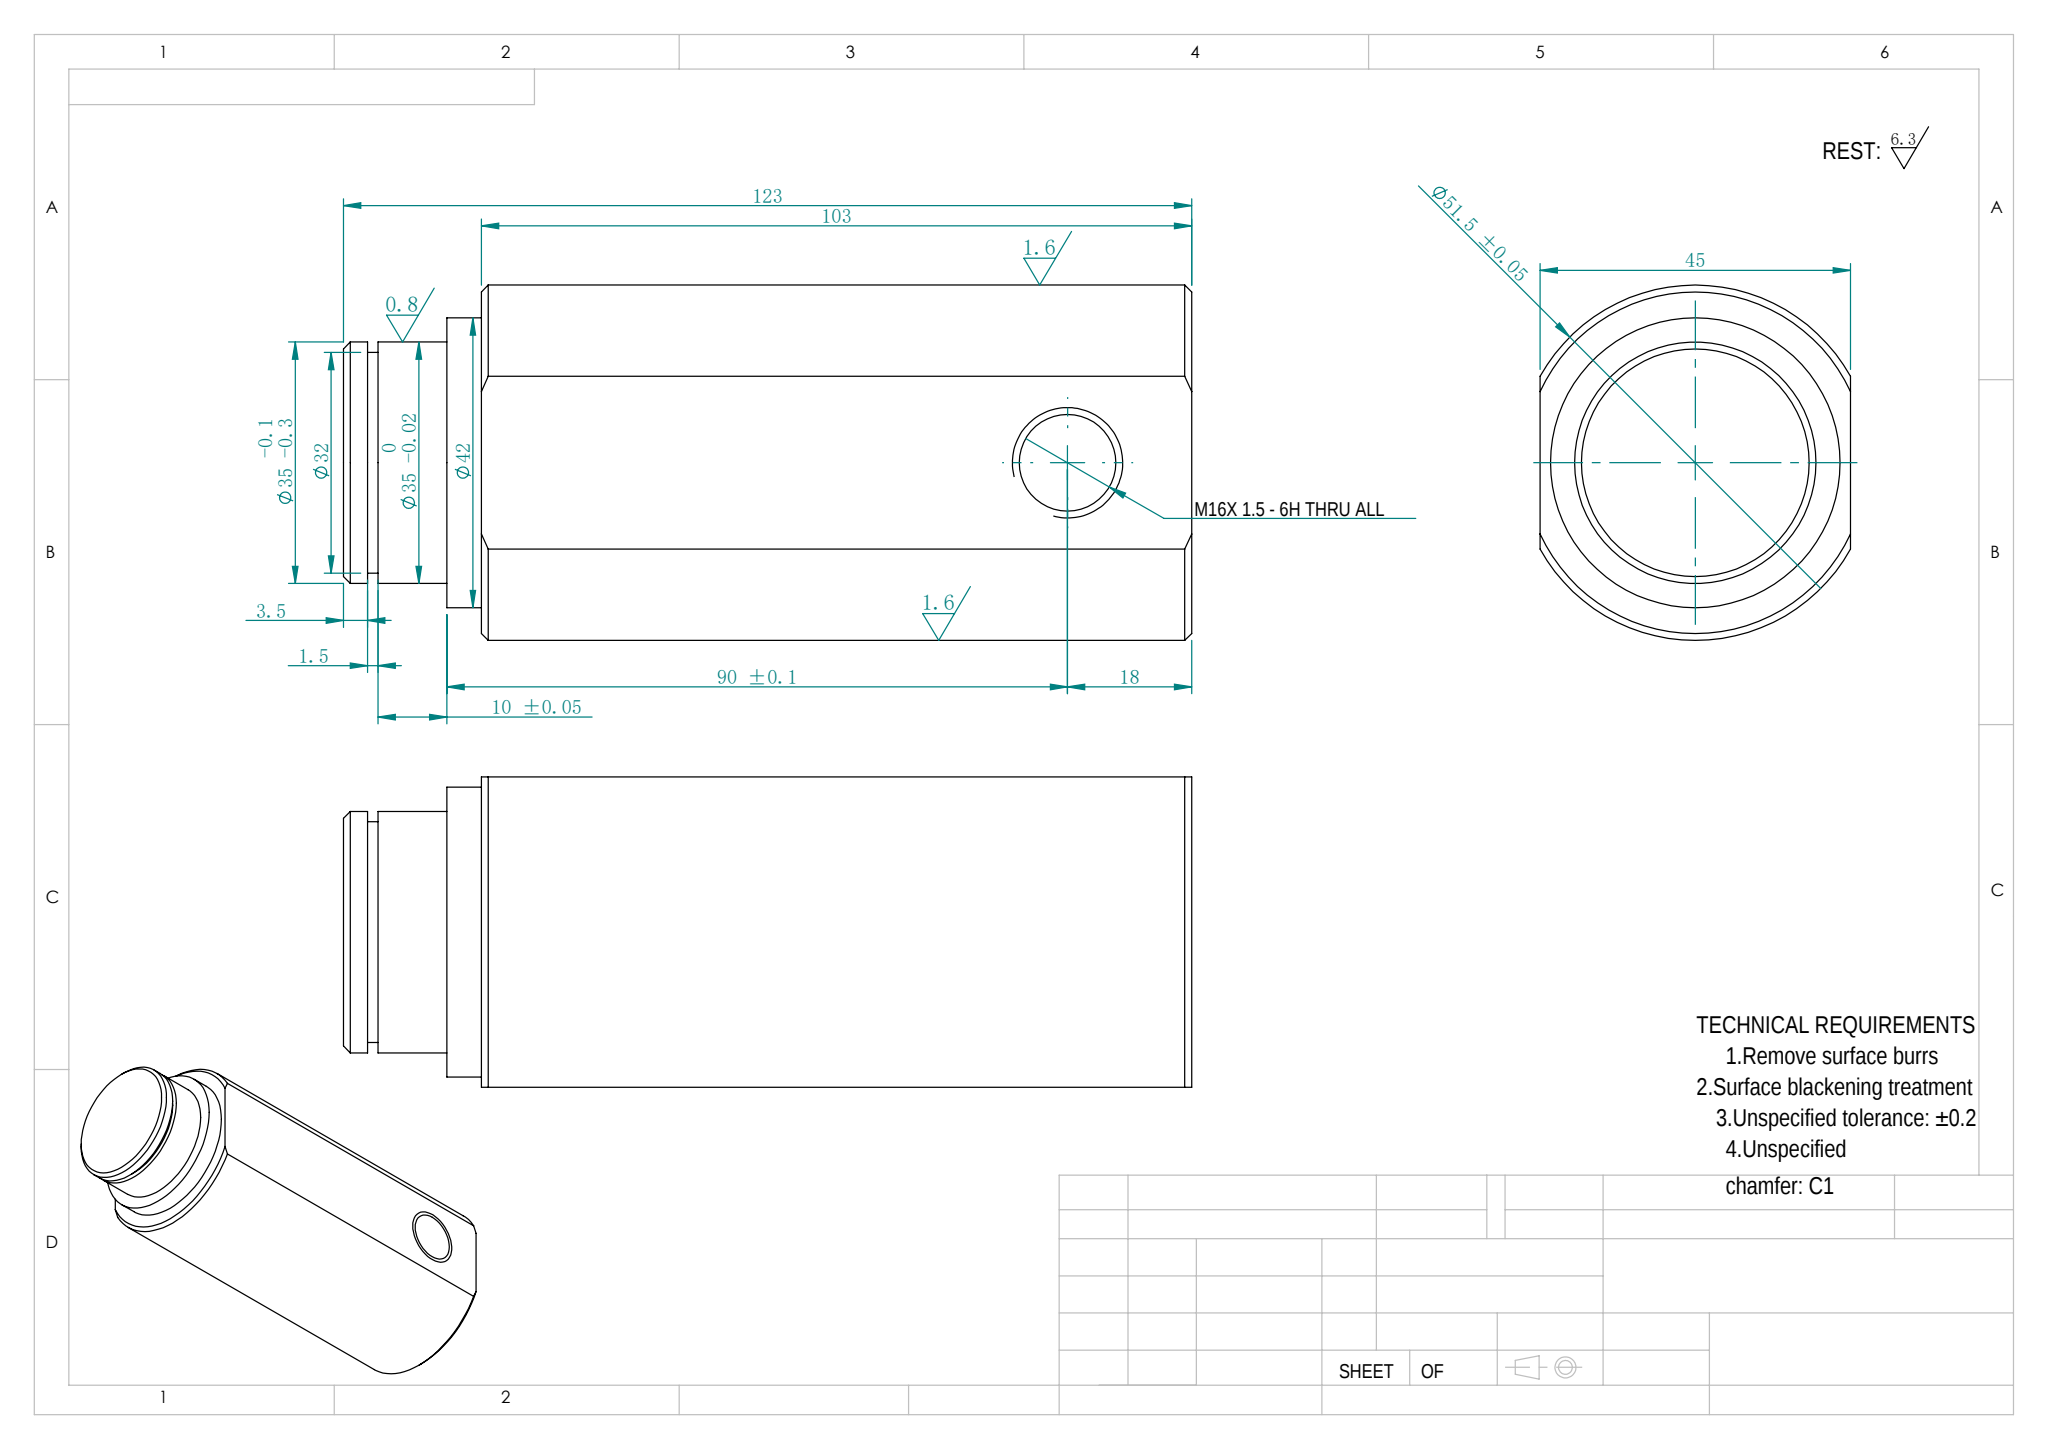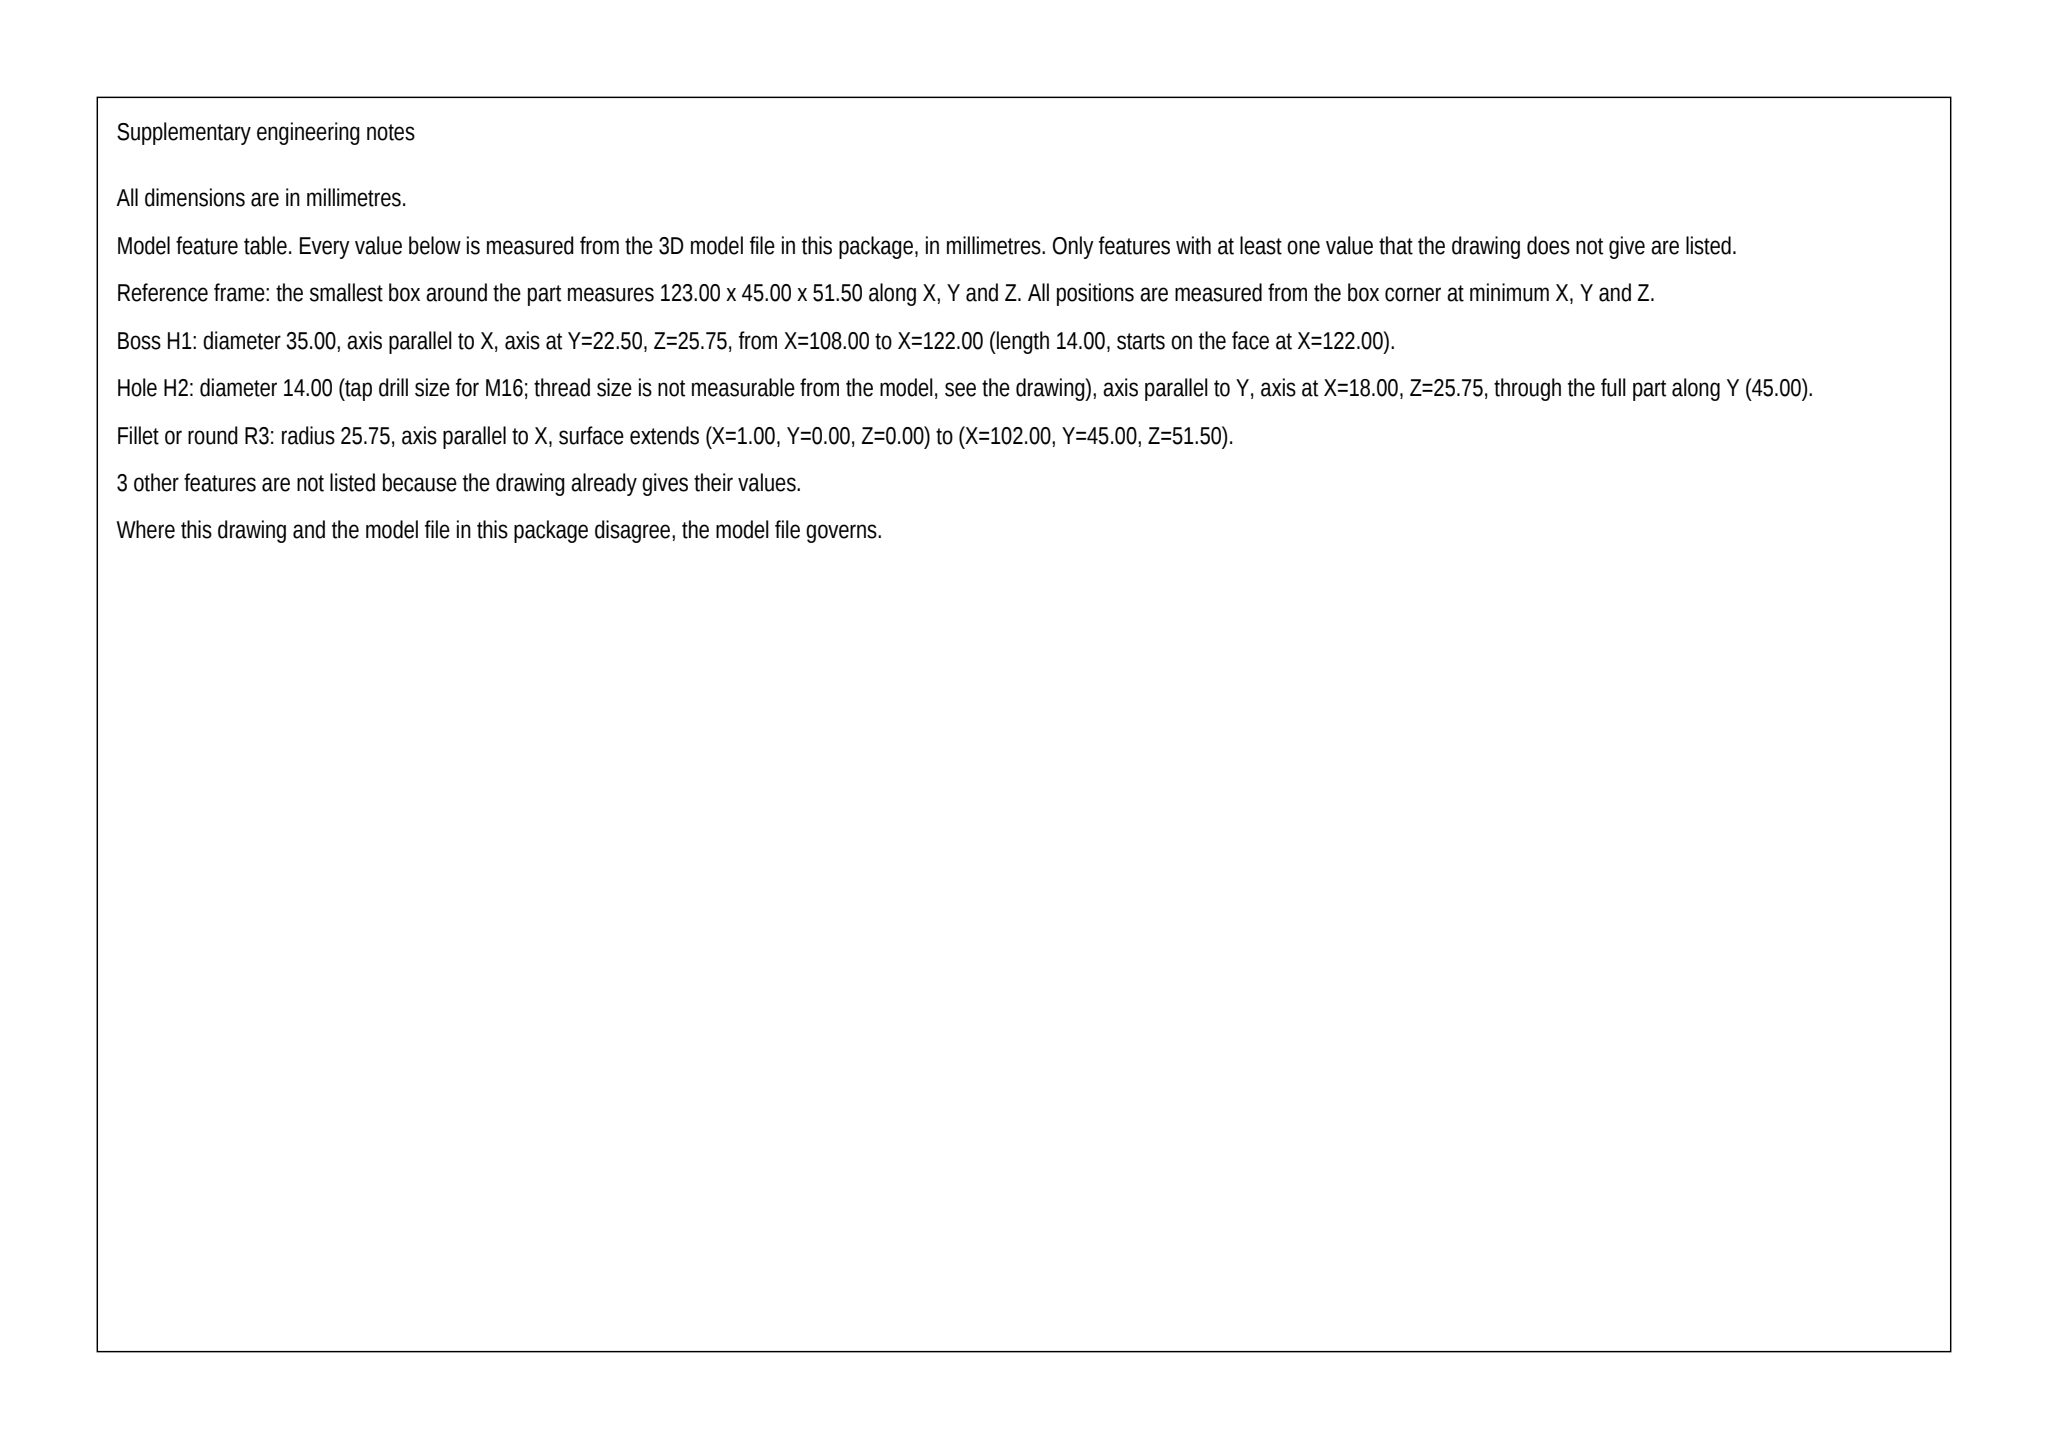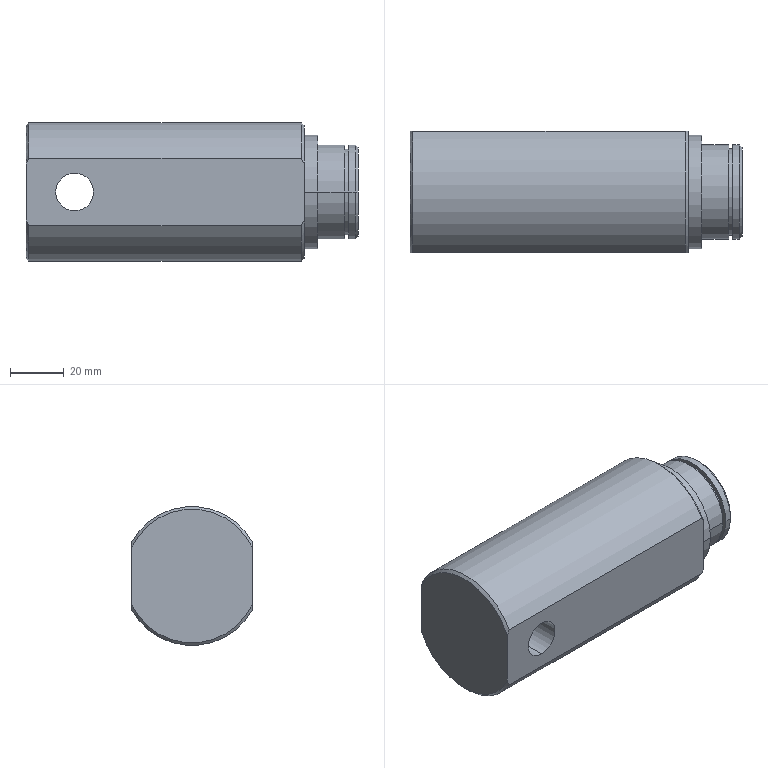Part | SolidWorks | mm | 1 solid | 26 faces | box 123 x 45 x 51.5 mm | volume 217259 mm3 | cylinder 12 | plane 8 | cone 6 | commonest cylinder face diameters 35 x4 14 x2 32 x2 42 x2 51.5 x2
build123d program:
from build123d import *

# Parameters (mm, degrees)
SKETCH2_OUTSIDE_W   = 82.09
SKETCH2_OUTSIDE_H   = 82.09
SKETCH2_OUTSIDE_W_2 = 65
SKETCH2_OUTSIDE_H_2 = 45
CUT_EXTRUDE1_DEPTH  = 129.278
M16_TAPPED_HOLE1_D  = 14
CHAMFER1_SIZE       = 1


with BuildPart() as part:
    # Sketch1 → Revolve1 (revolve)
    with BuildSketch(Plane.XY):
        Polygon((0, 0), (0, 25.75), (103, 25.75), (103, 21), (108, 21), (108, 17.5), (118, 17.5), (118, 16), (119.5, 16), (119.5, 17.5), (123, 17.5), (123, 0), align=None)
    revolve(axis=Axis((123, 0, 0), (-1, 0, 0)))

    # Sketch2 outside → Cut-Extrude1 (cut, through all)
    with BuildSketch(Plane.ZY):
        Rectangle(SKETCH2_OUTSIDE_W, SKETCH2_OUTSIDE_H)
        Rectangle(SKETCH2_OUTSIDE_W_2, SKETCH2_OUTSIDE_H_2, mode=Mode.SUBTRACT)
    extrude(amount=-CUT_EXTRUDE1_DEPTH, mode=Mode.SUBTRACT)

    # M16 Tapped Hole1 (through all)
    with Locations(Plane(origin=(0, 22.5, 0), x_dir=(1, 0, 0), z_dir=(0, 1, 0))):
        with Locations((18, 0)):
            Hole(M16_TAPPED_HOLE1_D / 2)

    # Chamfer1
    chamfer1_edges = [part.edges().sort_by_distance(p)[0] for p in [
        (103, 0, 25.75),
        (0, 0, 25.75),
        (103, 0, -25.75),
        (0, 0, -25.75),
        (123, -17.5, 0),
    ]]
    chamfer(chamfer1_edges, length=CHAMFER1_SIZE)


solid = part.part
STEP:
#1=CARTESIAN_POINT('',(123.,16.5,0.));
#2=VERTEX_POINT('',#1);
#3=CARTESIAN_POINT('',(123.,-16.5,0.));
#4=VERTEX_POINT('',#3);
#5=CARTESIAN_POINT('',(123.,0.,0.));
#6=DIRECTION('',(1.,0.,0.));
#7=DIRECTION('',(0.,1.,0.));
#8=AXIS2_PLACEMENT_3D('',#5,#6,#7);
#9=CIRCLE('',#8,16.5);
#10=EDGE_CURVE('',#2,#4,#9,.T.);
#11=ORIENTED_EDGE('',*,*,#10,.F.);
#12=CARTESIAN_POINT('',(122.,17.5,0.));
#13=VERTEX_POINT('',#12);
#14=CARTESIAN_POINT('',(123.,16.5,0.));
#15=DIRECTION('',(-0.7071,0.7071,0.));
#16=VECTOR('',#15,1000.);
#17=LINE('',#14,#16);
#18=EDGE_CURVE('',#2,#13,#17,.T.);
#19=ORIENTED_EDGE('',*,*,#18,.T.);
#20=CARTESIAN_POINT('',(122.,-17.5,0.));
#21=VERTEX_POINT('',#20);
#22=CARTESIAN_POINT('',(122.,0.,0.));
#23=DIRECTION('',(-1.,-0.,0.));
#24=DIRECTION('',(0.,1.,0.));
#25=AXIS2_PLACEMENT_3D('',#22,#23,#24);
#26=CIRCLE('',#25,17.5);
#27=EDGE_CURVE('',#21,#13,#26,.T.);
#28=ORIENTED_EDGE('',*,*,#27,.F.);
#29=CARTESIAN_POINT('',(123.,-16.5,0.));
#30=DIRECTION('',(-0.7071,-0.7071,0.));
#31=VECTOR('',#30,1000.);
#32=LINE('',#29,#31);
#33=EDGE_CURVE('',#4,#21,#32,.T.);
#34=ORIENTED_EDGE('',*,*,#33,.F.);
#35=EDGE_LOOP('',(#11,#19,#28,#34));
#36=FACE_OUTER_BOUND('',#35,.T.);
#37=CARTESIAN_POINT('',(123.,0.,0.));
#38=DIRECTION('',(-1.,-0.,0.));
#39=DIRECTION('',(0.,-1.,0.));
#40=AXIS2_PLACEMENT_3D('',#37,#38,#39);
#41=CONICAL_SURFACE('',#40,16.5,0.7854);
#42=ADVANCED_FACE('',(#36),#41,.T.);
#43=CARTESIAN_POINT('',(18.,-22.5,-7.));
#44=VERTEX_POINT('',#43);
#45=CARTESIAN_POINT('',(18.,-22.5,7.));
#46=VERTEX_POINT('',#45);
#47=CARTESIAN_POINT('',(18.,-22.5,0.));
#48=DIRECTION('',(0.,1.,0.));
#49=DIRECTION('',(0.,0.,1.));
#50=AXIS2_PLACEMENT_3D('',#47,#48,#49);
#51=CIRCLE('',#50,7.);
#52=EDGE_CURVE('',#44,#46,#51,.T.);
#53=ORIENTED_EDGE('',*,*,#52,.F.);
#54=CARTESIAN_POINT('',(18.,22.5,-7.));
#55=VERTEX_POINT('',#54);
#56=CARTESIAN_POINT('',(18.,22.5,-7.));
#57=DIRECTION('',(0.,1.,0.));
#58=VECTOR('',#57,1000.);
#59=LINE('',#56,#58);
#60=EDGE_CURVE('',#44,#55,#59,.T.);
#61=ORIENTED_EDGE('',*,*,#60,.T.);
#62=CARTESIAN_POINT('',(18.,22.5,7.));
#63=VERTEX_POINT('',#62);
#64=CARTESIAN_POINT('',(18.,22.5,0.));
#65=DIRECTION('',(0.,1.,0.));
#66=DIRECTION('',(0.,0.,1.));
#67=AXIS2_PLACEMENT_3D('',#64,#65,#66);
#68=CIRCLE('',#67,7.);
#69=EDGE_CURVE('',#55,#63,#68,.T.);
#70=ORIENTED_EDGE('',*,*,#69,.T.);
#71=CARTESIAN_POINT('',(18.,22.5,7.));
#72=DIRECTION('',(0.,1.,0.));
#73=VECTOR('',#72,1000.);
#74=LINE('',#71,#73);
#75=EDGE_CURVE('',#46,#63,#74,.T.);
#76=ORIENTED_EDGE('',*,*,#75,.F.);
#77=EDGE_LOOP('',(#53,#61,#70,#76));
#78=FACE_OUTER_BOUND('',#77,.T.);
#79=CARTESIAN_POINT('',(18.,22.5,0.));
#80=DIRECTION('',(0.,1.,0.));
#81=DIRECTION('',(0.,0.,1.));
#82=AXIS2_PLACEMENT_3D('',#79,#80,#81);
#83=CYLINDRICAL_SURFACE('',#82,7.);
#84=ADVANCED_FACE('',(#78),#83,.F.);
#85=CARTESIAN_POINT('',(119.5,17.5,0.));
#86=VERTEX_POINT('',#85);
#87=CARTESIAN_POINT('',(119.5,-17.5,0.));
#88=VERTEX_POINT('',#87);
#89=CARTESIAN_POINT('',(119.5,0.,0.));
#90=DIRECTION('',(1.,0.,0.));
#91=DIRECTION('',(0.,1.,0.));
#92=AXIS2_PLACEMENT_3D('',#89,#90,#91);
#93=CIRCLE('',#92,17.5);
#94=EDGE_CURVE('',#86,#88,#93,.T.);
#95=ORIENTED_EDGE('',*,*,#94,.T.);
#96=CARTESIAN_POINT('',(123.,-17.5,0.));
#97=DIRECTION('',(1.,0.,0.));
#98=VECTOR('',#97,1000.);
#99=LINE('',#96,#98);
#100=EDGE_CURVE('',#88,#21,#99,.T.);
#101=ORIENTED_EDGE('',*,*,#100,.T.);
#102=ORIENTED_EDGE('',*,*,#27,.T.);
#103=CARTESIAN_POINT('',(123.,17.5,0.));
#104=DIRECTION('',(1.,0.,0.));
#105=VECTOR('',#104,1000.);
#106=LINE('',#103,#105);
#107=EDGE_CURVE('',#86,#13,#106,.T.);
#108=ORIENTED_EDGE('',*,*,#107,.F.);
#109=EDGE_LOOP('',(#95,#101,#102,#108));
#110=FACE_OUTER_BOUND('',#109,.T.);
#111=CARTESIAN_POINT('',(123.,0.,0.));
#112=DIRECTION('',(1.,0.,0.));
#113=DIRECTION('',(0.,1.,0.));
#114=AXIS2_PLACEMENT_3D('',#111,#112,#113);
#115=CYLINDRICAL_SURFACE('',#114,17.5);
#116=ADVANCED_FACE('',(#110),#115,.T.);
#117=CARTESIAN_POINT('',(118.,16.,0.));
#118=VERTEX_POINT('',#117);
#119=CARTESIAN_POINT('',(118.,-16.,0.));
#120=VERTEX_POINT('',#119);
#121=CARTESIAN_POINT('',(118.,0.,0.));
#122=DIRECTION('',(1.,0.,0.));
#123=DIRECTION('',(0.,1.,0.));
#124=AXIS2_PLACEMENT_3D('',#121,#122,#123);
#125=CIRCLE('',#124,16.);
#126=EDGE_CURVE('',#118,#120,#125,.T.);
#127=ORIENTED_EDGE('',*,*,#126,.T.);
#128=CARTESIAN_POINT('',(119.5,-16.,0.));
#129=VERTEX_POINT('',#128);
#130=CARTESIAN_POINT('',(123.,-16.,0.));
#131=DIRECTION('',(1.,0.,0.));
#132=VECTOR('',#131,1000.);
#133=LINE('',#130,#132);
#134=EDGE_CURVE('',#120,#129,#133,.T.);
#135=ORIENTED_EDGE('',*,*,#134,.T.);
#136=CARTESIAN_POINT('',(119.5,16.,0.));
#137=VERTEX_POINT('',#136);
#138=CARTESIAN_POINT('',(119.5,0.,0.));
#139=DIRECTION('',(1.,0.,0.));
#140=DIRECTION('',(0.,1.,0.));
#141=AXIS2_PLACEMENT_3D('',#138,#139,#140);
#142=CIRCLE('',#141,16.);
#143=EDGE_CURVE('',#137,#129,#142,.T.);
#144=ORIENTED_EDGE('',*,*,#143,.F.);
#145=CARTESIAN_POINT('',(123.,16.,0.));
#146=DIRECTION('',(1.,0.,0.));
#147=VECTOR('',#146,1000.);
#148=LINE('',#145,#147);
#149=EDGE_CURVE('',#118,#137,#148,.T.);
#150=ORIENTED_EDGE('',*,*,#149,.F.);
#151=EDGE_LOOP('',(#127,#135,#144,#150));
#152=FACE_OUTER_BOUND('',#151,.T.);
#153=CARTESIAN_POINT('',(123.,0.,0.));
#154=DIRECTION('',(1.,0.,0.));
#155=DIRECTION('',(0.,1.,0.));
#156=AXIS2_PLACEMENT_3D('',#153,#154,#155);
#157=CYLINDRICAL_SURFACE('',#156,16.);
#158=ADVANCED_FACE('',(#152),#157,.T.);
#159=CARTESIAN_POINT('',(108.,17.5,0.));
#160=VERTEX_POINT('',#159);
#161=CARTESIAN_POINT('',(108.,-17.5,0.));
#162=VERTEX_POINT('',#161);
#163=CARTESIAN_POINT('',(108.,0.,0.));
#164=DIRECTION('',(1.,0.,0.));
#165=DIRECTION('',(0.,1.,0.));
#166=AXIS2_PLACEMENT_3D('',#163,#164,#165);
#167=CIRCLE('',#166,17.5);
#168=EDGE_CURVE('',#160,#162,#167,.T.);
#169=ORIENTED_EDGE('',*,*,#168,.T.);
#170=CARTESIAN_POINT('',(118.,-17.5,0.));
#171=VERTEX_POINT('',#170);
#172=CARTESIAN_POINT('',(123.,-17.5,0.));
#173=DIRECTION('',(1.,0.,0.));
#174=VECTOR('',#173,1000.);
#175=LINE('',#172,#174);
#176=EDGE_CURVE('',#162,#171,#175,.T.);
#177=ORIENTED_EDGE('',*,*,#176,.T.);
#178=CARTESIAN_POINT('',(118.,17.5,0.));
#179=VERTEX_POINT('',#178);
#180=CARTESIAN_POINT('',(118.,0.,0.));
#181=DIRECTION('',(1.,0.,0.));
#182=DIRECTION('',(0.,1.,0.));
#183=AXIS2_PLACEMENT_3D('',#180,#181,#182);
#184=CIRCLE('',#183,17.5);
#185=EDGE_CURVE('',#179,#171,#184,.T.);
#186=ORIENTED_EDGE('',*,*,#185,.F.);
#187=CARTESIAN_POINT('',(123.,17.5,0.));
#188=DIRECTION('',(1.,0.,0.));
#189=VECTOR('',#188,1000.);
#190=LINE('',#187,#189);
#191=EDGE_CURVE('',#160,#179,#190,.T.);
#192=ORIENTED_EDGE('',*,*,#191,.F.);
#193=EDGE_LOOP('',(#169,#177,#186,#192));
#194=FACE_OUTER_BOUND('',#193,.T.);
#195=CARTESIAN_POINT('',(123.,0.,0.));
#196=DIRECTION('',(1.,0.,0.));
#197=DIRECTION('',(0.,1.,0.));
#198=AXIS2_PLACEMENT_3D('',#195,#196,#197);
#199=CYLINDRICAL_SURFACE('',#198,17.5);
#200=ADVANCED_FACE('',(#194),#199,.T.);
#201=CARTESIAN_POINT('',(103.,21.,0.));
#202=VERTEX_POINT('',#201);
#203=CARTESIAN_POINT('',(103.,-21.,0.));
#204=VERTEX_POINT('',#203);
#205=CARTESIAN_POINT('',(103.,0.,0.));
#206=DIRECTION('',(1.,0.,0.));
#207=DIRECTION('',(0.,1.,0.));
#208=AXIS2_PLACEMENT_3D('',#205,#206,#207);
#209=CIRCLE('',#208,21.);
#210=EDGE_CURVE('',#202,#204,#209,.T.);
#211=ORIENTED_EDGE('',*,*,#210,.T.);
#212=CARTESIAN_POINT('',(108.,-21.,0.));
#213=VERTEX_POINT('',#212);
#214=CARTESIAN_POINT('',(123.,-21.,0.));
#215=DIRECTION('',(1.,0.,0.));
#216=VECTOR('',#215,1000.);
#217=LINE('',#214,#216);
#218=EDGE_CURVE('',#204,#213,#217,.T.);
#219=ORIENTED_EDGE('',*,*,#218,.T.);
#220=CARTESIAN_POINT('',(108.,21.,0.));
#221=VERTEX_POINT('',#220);
#222=CARTESIAN_POINT('',(108.,0.,0.));
#223=DIRECTION('',(1.,0.,0.));
#224=DIRECTION('',(0.,1.,0.));
#225=AXIS2_PLACEMENT_3D('',#222,#223,#224);
#226=CIRCLE('',#225,21.);
#227=EDGE_CURVE('',#221,#213,#226,.T.);
#228=ORIENTED_EDGE('',*,*,#227,.F.);
#229=CARTESIAN_POINT('',(123.,21.,0.));
#230=DIRECTION('',(1.,0.,0.));
#231=VECTOR('',#230,1000.);
#232=LINE('',#229,#231);
#233=EDGE_CURVE('',#202,#221,#232,.T.);
#234=ORIENTED_EDGE('',*,*,#233,.F.);
#235=EDGE_LOOP('',(#211,#219,#228,#234));
#236=FACE_OUTER_BOUND('',#235,.T.);
#237=CARTESIAN_POINT('',(123.,0.,0.));
#238=DIRECTION('',(1.,0.,0.));
#239=DIRECTION('',(0.,1.,0.));
#240=AXIS2_PLACEMENT_3D('',#237,#238,#239);
#241=CYLINDRICAL_SURFACE('',#240,21.);
#242=ADVANCED_FACE('',(#236),#241,.T.);
#243=CARTESIAN_POINT('',(0.,-22.5,-10.311));
#244=VERTEX_POINT('',#243);
#245=CARTESIAN_POINT('',(0.,-22.5,10.311));
#246=VERTEX_POINT('',#245);
#247=CARTESIAN_POINT('',(0.,-22.5,-32.5));
#248=DIRECTION('',(0.,0.,1.));
#249=VECTOR('',#248,1000.);
#250=LINE('',#247,#249);
#251=EDGE_CURVE('',#244,#246,#250,.T.);
#252=ORIENTED_EDGE('',*,*,#251,.T.);
#253=CARTESIAN_POINT('',(-0.,22.5,10.311));
#254=VERTEX_POINT('',#253);
#255=CARTESIAN_POINT('',(0.,0.,0.));
#256=DIRECTION('',(-1.,-0.,0.));
#257=DIRECTION('',(0.,-1.,0.));
#258=AXIS2_PLACEMENT_3D('',#255,#256,#257);
#259=CIRCLE('',#258,24.75);
#260=EDGE_CURVE('',#246,#254,#259,.T.);
#261=ORIENTED_EDGE('',*,*,#260,.T.);
#262=CARTESIAN_POINT('',(-0.,22.5,-10.311));
#263=VERTEX_POINT('',#262);
#264=CARTESIAN_POINT('',(-0.,22.5,-32.5));
#265=DIRECTION('',(0.,0.,-1.));
#266=VECTOR('',#265,1000.);
#267=LINE('',#264,#266);
#268=EDGE_CURVE('',#254,#263,#267,.T.);
#269=ORIENTED_EDGE('',*,*,#268,.T.);
#270=CARTESIAN_POINT('',(0.,0.,0.));
#271=DIRECTION('',(-1.,-0.,0.));
#272=DIRECTION('',(0.,-1.,0.));
#273=AXIS2_PLACEMENT_3D('',#270,#271,#272);
#274=CIRCLE('',#273,24.75);
#275=EDGE_CURVE('',#263,#244,#274,.T.);
#276=ORIENTED_EDGE('',*,*,#275,.T.);
#277=EDGE_LOOP('',(#252,#261,#269,#276));
#278=FACE_OUTER_BOUND('',#277,.T.);
#279=CARTESIAN_POINT('',(0.,0.,0.));
#280=DIRECTION('',(-1.,-0.,0.));
#281=DIRECTION('',(0.,-1.,0.));
#282=AXIS2_PLACEMENT_3D('',#279,#280,#281);
#283=PLANE('',#282);
#284=ADVANCED_FACE('',(#278),#283,.T.);
#285=CARTESIAN_POINT('',(102.,-22.5,-12.522));
#286=VERTEX_POINT('',#285);
#287=CARTESIAN_POINT('',(1.,-22.5,-12.522));
#288=VERTEX_POINT('',#287);
#289=CARTESIAN_POINT('',(123.,-22.5,-12.522));
#290=DIRECTION('',(-1.,-0.,0.));
#291=VECTOR('',#290,1000.);
#292=LINE('',#289,#291);
#293=EDGE_CURVE('',#286,#288,#292,.T.);
#294=ORIENTED_EDGE('',*,*,#293,.T.);
#295=CARTESIAN_POINT('',(1.,22.5,-12.522));
#296=VERTEX_POINT('',#295);
#297=CARTESIAN_POINT('',(1.,0.,0.));
#298=DIRECTION('',(1.,0.,0.));
#299=DIRECTION('',(0.,-1.,0.));
#300=AXIS2_PLACEMENT_3D('',#297,#298,#299);
#301=CIRCLE('',#300,25.75);
#302=EDGE_CURVE('',#288,#296,#301,.T.);
#303=ORIENTED_EDGE('',*,*,#302,.T.);
#304=CARTESIAN_POINT('',(102.,22.5,-12.522));
#305=VERTEX_POINT('',#304);
#306=CARTESIAN_POINT('',(123.,22.5,-12.522));
#307=DIRECTION('',(1.,0.,0.));
#308=VECTOR('',#307,1000.);
#309=LINE('',#306,#308);
#310=EDGE_CURVE('',#296,#305,#309,.T.);
#311=ORIENTED_EDGE('',*,*,#310,.T.);
#312=CARTESIAN_POINT('',(102.,0.,0.));
#313=DIRECTION('',(-1.,-0.,0.));
#314=DIRECTION('',(0.,1.,0.));
#315=AXIS2_PLACEMENT_3D('',#312,#313,#314);
#316=CIRCLE('',#315,25.75);
#317=EDGE_CURVE('',#305,#286,#316,.T.);
#318=ORIENTED_EDGE('',*,*,#317,.T.);
#319=EDGE_LOOP('',(#294,#303,#311,#318));
#320=FACE_OUTER_BOUND('',#319,.T.);
#321=CARTESIAN_POINT('',(123.,0.,0.));
#322=DIRECTION('',(1.,0.,0.));
#323=DIRECTION('',(0.,1.,0.));
#324=AXIS2_PLACEMENT_3D('',#321,#322,#323);
#325=CYLINDRICAL_SURFACE('',#324,25.75);
#326=ADVANCED_FACE('',(#320),#325,.T.);
#327=CARTESIAN_POINT('',(102.,22.5,12.522));
#328=VERTEX_POINT('',#327);
#329=CARTESIAN_POINT('',(1.,22.5,12.522));
#330=VERTEX_POINT('',#329);
#331=CARTESIAN_POINT('',(123.,22.5,12.522));
#332=DIRECTION('',(-1.,-0.,0.));
#333=VECTOR('',#332,1000.);
#334=LINE('',#331,#333);
#335=EDGE_CURVE('',#328,#330,#334,.T.);
#336=ORIENTED_EDGE('',*,*,#335,.T.);
#337=CARTESIAN_POINT('',(1.,-22.5,12.522));
#338=VERTEX_POINT('',#337);
#339=CARTESIAN_POINT('',(1.,0.,0.));
#340=DIRECTION('',(1.,0.,0.));
#341=DIRECTION('',(0.,-1.,0.));
#342=AXIS2_PLACEMENT_3D('',#339,#340,#341);
#343=CIRCLE('',#342,25.75);
#344=EDGE_CURVE('',#330,#338,#343,.T.);
#345=ORIENTED_EDGE('',*,*,#344,.T.);
#346=CARTESIAN_POINT('',(102.,-22.5,12.522));
#347=VERTEX_POINT('',#346);
#348=CARTESIAN_POINT('',(123.,-22.5,12.522));
#349=DIRECTION('',(1.,0.,0.));
#350=VECTOR('',#349,1000.);
#351=LINE('',#348,#350);
#352=EDGE_CURVE('',#338,#347,#351,.T.);
#353=ORIENTED_EDGE('',*,*,#352,.T.);
#354=CARTESIAN_POINT('',(102.,0.,0.));
#355=DIRECTION('',(-1.,-0.,0.));
#356=DIRECTION('',(0.,1.,0.));
#357=AXIS2_PLACEMENT_3D('',#354,#355,#356);
#358=CIRCLE('',#357,25.75);
#359=EDGE_CURVE('',#347,#328,#358,.T.);
#360=ORIENTED_EDGE('',*,*,#359,.T.);
#361=EDGE_LOOP('',(#336,#345,#353,#360));
#362=FACE_OUTER_BOUND('',#361,.T.);
#363=CARTESIAN_POINT('',(123.,0.,0.));
#364=DIRECTION('',(1.,0.,0.));
#365=DIRECTION('',(0.,1.,0.));
#366=AXIS2_PLACEMENT_3D('',#363,#364,#365);
#367=CYLINDRICAL_SURFACE('',#366,25.75);
#368=ADVANCED_FACE('',(#362),#367,.T.);
#369=ORIENTED_EDGE('',*,*,#210,.F.);
#370=CARTESIAN_POINT('',(103.,0.,0.));
#371=DIRECTION('',(1.,0.,0.));
#372=DIRECTION('',(0.,1.,0.));
#373=AXIS2_PLACEMENT_3D('',#370,#371,#372);
#374=CIRCLE('',#373,21.);
#375=EDGE_CURVE('',#204,#202,#374,.T.);
#376=ORIENTED_EDGE('',*,*,#375,.F.);
#377=EDGE_LOOP('',(#369,#376));
#378=FACE_BOUND('',#377,.T.);
#379=CARTESIAN_POINT('',(103.,-22.5,10.311));
#380=VERTEX_POINT('',#379);
#381=CARTESIAN_POINT('',(103.,-22.5,-10.311));
#382=VERTEX_POINT('',#381);
#383=CARTESIAN_POINT('',(103.,-22.5,0.));
#384=DIRECTION('',(0.,0.,-1.));
#385=VECTOR('',#384,1000.);
#386=LINE('',#383,#385);
#387=EDGE_CURVE('',#380,#382,#386,.T.);
#388=ORIENTED_EDGE('',*,*,#387,.T.);
#389=CARTESIAN_POINT('',(103.,22.5,-10.311));
#390=VERTEX_POINT('',#389);
#391=CARTESIAN_POINT('',(103.,0.,0.));
#392=DIRECTION('',(1.,0.,0.));
#393=DIRECTION('',(0.,1.,0.));
#394=AXIS2_PLACEMENT_3D('',#391,#392,#393);
#395=CIRCLE('',#394,24.75);
#396=EDGE_CURVE('',#382,#390,#395,.T.);
#397=ORIENTED_EDGE('',*,*,#396,.T.);
#398=CARTESIAN_POINT('',(103.,22.5,10.311));
#399=VERTEX_POINT('',#398);
#400=CARTESIAN_POINT('',(103.,22.5,0.));
#401=DIRECTION('',(0.,0.,1.));
#402=VECTOR('',#401,1000.);
#403=LINE('',#400,#402);
#404=EDGE_CURVE('',#390,#399,#403,.T.);
#405=ORIENTED_EDGE('',*,*,#404,.T.);
#406=CARTESIAN_POINT('',(103.,0.,0.));
#407=DIRECTION('',(1.,0.,0.));
#408=DIRECTION('',(0.,1.,0.));
#409=AXIS2_PLACEMENT_3D('',#406,#407,#408);
#410=CIRCLE('',#409,24.75);
#411=EDGE_CURVE('',#399,#380,#410,.T.);
#412=ORIENTED_EDGE('',*,*,#411,.T.);
#413=EDGE_LOOP('',(#388,#397,#405,#412));
#414=FACE_OUTER_BOUND('',#413,.T.);
#415=CARTESIAN_POINT('',(103.,25.75,0.));
#416=DIRECTION('',(1.,0.,0.));
#417=DIRECTION('',(-0.,1.,0.));
#418=AXIS2_PLACEMENT_3D('',#415,#416,#417);
#419=PLANE('',#418);
#420=ADVANCED_FACE('',(#378,#414),#419,.T.);
#421=ORIENTED_EDGE('',*,*,#218,.F.);
#422=ORIENTED_EDGE('',*,*,#375,.T.);
#423=ORIENTED_EDGE('',*,*,#233,.T.);
#424=CARTESIAN_POINT('',(108.,0.,0.));
#425=DIRECTION('',(1.,0.,0.));
#426=DIRECTION('',(0.,1.,0.));
#427=AXIS2_PLACEMENT_3D('',#424,#425,#426);
#428=CIRCLE('',#427,21.);
#429=EDGE_CURVE('',#213,#221,#428,.T.);
#430=ORIENTED_EDGE('',*,*,#429,.F.);
#431=EDGE_LOOP('',(#421,#422,#423,#430));
#432=FACE_OUTER_BOUND('',#431,.T.);
#433=CARTESIAN_POINT('',(123.,0.,0.));
#434=DIRECTION('',(1.,0.,0.));
#435=DIRECTION('',(0.,1.,0.));
#436=AXIS2_PLACEMENT_3D('',#433,#434,#435);
#437=CYLINDRICAL_SURFACE('',#436,21.);
#438=ADVANCED_FACE('',(#432),#437,.T.);
#439=ORIENTED_EDGE('',*,*,#227,.T.);
#440=ORIENTED_EDGE('',*,*,#429,.T.);
#441=EDGE_LOOP('',(#439,#440));
#442=FACE_OUTER_BOUND('',#441,.T.);
#443=ORIENTED_EDGE('',*,*,#168,.F.);
#444=CARTESIAN_POINT('',(108.,0.,0.));
#445=DIRECTION('',(1.,0.,0.));
#446=DIRECTION('',(0.,1.,0.));
#447=AXIS2_PLACEMENT_3D('',#444,#445,#446);
#448=CIRCLE('',#447,17.5);
#449=EDGE_CURVE('',#162,#160,#448,.T.);
#450=ORIENTED_EDGE('',*,*,#449,.F.);
#451=EDGE_LOOP('',(#443,#450));
#452=FACE_BOUND('',#451,.T.);
#453=CARTESIAN_POINT('',(108.,21.,0.));
#454=DIRECTION('',(1.,0.,0.));
#455=DIRECTION('',(-0.,1.,0.));
#456=AXIS2_PLACEMENT_3D('',#453,#454,#455);
#457=PLANE('',#456);
#458=ADVANCED_FACE('',(#442,#452),#457,.T.);
#459=ORIENTED_EDGE('',*,*,#176,.F.);
#460=ORIENTED_EDGE('',*,*,#449,.T.);
#461=ORIENTED_EDGE('',*,*,#191,.T.);
#462=CARTESIAN_POINT('',(118.,0.,0.));
#463=DIRECTION('',(1.,0.,0.));
#464=DIRECTION('',(0.,1.,0.));
#465=AXIS2_PLACEMENT_3D('',#462,#463,#464);
#466=CIRCLE('',#465,17.5);
#467=EDGE_CURVE('',#171,#179,#466,.T.);
#468=ORIENTED_EDGE('',*,*,#467,.F.);
#469=EDGE_LOOP('',(#459,#460,#461,#468));
#470=FACE_OUTER_BOUND('',#469,.T.);
#471=CARTESIAN_POINT('',(123.,0.,0.));
#472=DIRECTION('',(1.,0.,0.));
#473=DIRECTION('',(0.,1.,0.));
#474=AXIS2_PLACEMENT_3D('',#471,#472,#473);
#475=CYLINDRICAL_SURFACE('',#474,17.5);
#476=ADVANCED_FACE('',(#470),#475,.T.);
#477=ORIENTED_EDGE('',*,*,#185,.T.);
#478=ORIENTED_EDGE('',*,*,#467,.T.);
#479=EDGE_LOOP('',(#477,#478));
#480=FACE_OUTER_BOUND('',#479,.T.);
#481=ORIENTED_EDGE('',*,*,#126,.F.);
#482=CARTESIAN_POINT('',(118.,0.,0.));
#483=DIRECTION('',(1.,0.,0.));
#484=DIRECTION('',(0.,1.,0.));
#485=AXIS2_PLACEMENT_3D('',#482,#483,#484);
#486=CIRCLE('',#485,16.);
#487=EDGE_CURVE('',#120,#118,#486,.T.);
#488=ORIENTED_EDGE('',*,*,#487,.F.);
#489=EDGE_LOOP('',(#481,#488));
#490=FACE_BOUND('',#489,.T.);
#491=CARTESIAN_POINT('',(118.,17.5,0.));
#492=DIRECTION('',(1.,0.,0.));
#493=DIRECTION('',(-0.,1.,0.));
#494=AXIS2_PLACEMENT_3D('',#491,#492,#493);
#495=PLANE('',#494);
#496=ADVANCED_FACE('',(#480,#490),#495,.T.);
#497=ORIENTED_EDGE('',*,*,#134,.F.);
#498=ORIENTED_EDGE('',*,*,#487,.T.);
#499=ORIENTED_EDGE('',*,*,#149,.T.);
#500=CARTESIAN_POINT('',(119.5,0.,0.));
#501=DIRECTION('',(1.,0.,0.));
#502=DIRECTION('',(0.,1.,0.));
#503=AXIS2_PLACEMENT_3D('',#500,#501,#502);
#504=CIRCLE('',#503,16.);
#505=EDGE_CURVE('',#129,#137,#504,.T.);
#506=ORIENTED_EDGE('',*,*,#505,.F.);
#507=EDGE_LOOP('',(#497,#498,#499,#506));
#508=FACE_OUTER_BOUND('',#507,.T.);
#509=CARTESIAN_POINT('',(123.,0.,0.));
#510=DIRECTION('',(1.,0.,0.));
#511=DIRECTION('',(0.,1.,0.));
#512=AXIS2_PLACEMENT_3D('',#509,#510,#511);
#513=CYLINDRICAL_SURFACE('',#512,16.);
#514=ADVANCED_FACE('',(#508),#513,.T.);
#515=ORIENTED_EDGE('',*,*,#143,.T.);
#516=ORIENTED_EDGE('',*,*,#505,.T.);
#517=EDGE_LOOP('',(#515,#516));
#518=FACE_BOUND('',#517,.T.);
#519=ORIENTED_EDGE('',*,*,#94,.F.);
#520=CARTESIAN_POINT('',(119.5,0.,0.));
#521=DIRECTION('',(1.,0.,0.));
#522=DIRECTION('',(0.,1.,0.));
#523=AXIS2_PLACEMENT_3D('',#520,#521,#522);
#524=CIRCLE('',#523,17.5);
#525=EDGE_CURVE('',#88,#86,#524,.T.);
#526=ORIENTED_EDGE('',*,*,#525,.F.);
#527=EDGE_LOOP('',(#519,#526));
#528=FACE_OUTER_BOUND('',#527,.T.);
#529=CARTESIAN_POINT('',(119.5,17.5,0.));
#530=DIRECTION('',(-1.,-0.,0.));
#531=DIRECTION('',(0.,-1.,0.));
#532=AXIS2_PLACEMENT_3D('',#529,#530,#531);
#533=PLANE('',#532);
#534=ADVANCED_FACE('',(#518,#528),#533,.T.);
#535=ORIENTED_EDGE('',*,*,#100,.F.);
#536=ORIENTED_EDGE('',*,*,#525,.T.);
#537=ORIENTED_EDGE('',*,*,#107,.T.);
#538=CARTESIAN_POINT('',(122.,0.,0.));
#539=DIRECTION('',(-1.,-0.,0.));
#540=DIRECTION('',(0.,1.,0.));
#541=AXIS2_PLACEMENT_3D('',#538,#539,#540);
#542=CIRCLE('',#541,17.5);
#543=EDGE_CURVE('',#13,#21,#542,.T.);
#544=ORIENTED_EDGE('',*,*,#543,.T.);
#545=EDGE_LOOP('',(#535,#536,#537,#544));
#546=FACE_OUTER_BOUND('',#545,.T.);
#547=CARTESIAN_POINT('',(123.,0.,0.));
#548=DIRECTION('',(1.,0.,0.));
#549=DIRECTION('',(0.,1.,0.));
#550=AXIS2_PLACEMENT_3D('',#547,#548,#549);
#551=CYLINDRICAL_SURFACE('',#550,17.5);
#552=ADVANCED_FACE('',(#546),#551,.T.);
#553=CARTESIAN_POINT('',(123.,0.,0.));
#554=DIRECTION('',(1.,0.,0.));
#555=DIRECTION('',(0.,1.,0.));
#556=AXIS2_PLACEMENT_3D('',#553,#554,#555);
#557=CIRCLE('',#556,16.5);
#558=EDGE_CURVE('',#4,#2,#557,.T.);
#559=ORIENTED_EDGE('',*,*,#558,.T.);
#560=ORIENTED_EDGE('',*,*,#10,.T.);
#561=EDGE_LOOP('',(#559,#560));
#562=FACE_OUTER_BOUND('',#561,.T.);
#563=CARTESIAN_POINT('',(123.,17.5,0.));
#564=DIRECTION('',(1.,0.,0.));
#565=DIRECTION('',(-0.,1.,0.));
#566=AXIS2_PLACEMENT_3D('',#563,#564,#565);
#567=PLANE('',#566);
#568=ADVANCED_FACE('',(#562),#567,.T.);
#569=CARTESIAN_POINT('',(18.,22.5,0.));
#570=DIRECTION('',(0.,1.,0.));
#571=DIRECTION('',(0.,0.,1.));
#572=AXIS2_PLACEMENT_3D('',#569,#570,#571);
#573=CIRCLE('',#572,7.);
#574=EDGE_CURVE('',#63,#55,#573,.T.);
#575=ORIENTED_EDGE('',*,*,#574,.F.);
#576=ORIENTED_EDGE('',*,*,#69,.F.);
#577=EDGE_LOOP('',(#575,#576));
#578=FACE_BOUND('',#577,.T.);
#579=ORIENTED_EDGE('',*,*,#268,.F.);
#580=CARTESIAN_POINT('',(-0.,22.5,10.311));
#581=CARTESIAN_POINT('',(0.3113,22.5,11.058));
#582=CARTESIAN_POINT('',(0.646,22.5,11.795));
#583=CARTESIAN_POINT('',(1.,22.5,12.522));
#584=B_SPLINE_CURVE_WITH_KNOTS('',3,(#580,#581,#582,#583),.UNSPECIFIED.,.F.,.F.,(4,4),(0.,0.002427),.UNSPECIFIED.);
#585=EDGE_CURVE('',#254,#330,#584,.T.);
#586=ORIENTED_EDGE('',*,*,#585,.T.);
#587=ORIENTED_EDGE('',*,*,#335,.F.);
#588=CARTESIAN_POINT('',(102.,22.5,12.522));
#589=CARTESIAN_POINT('',(102.354,22.5,11.795));
#590=CARTESIAN_POINT('',(102.689,22.5,11.058));
#591=CARTESIAN_POINT('',(103.,22.5,10.311));
#592=B_SPLINE_CURVE_WITH_KNOTS('',3,(#588,#589,#590,#591),.UNSPECIFIED.,.F.,.F.,(4,4),(0.,0.002427),.UNSPECIFIED.);
#593=EDGE_CURVE('',#328,#399,#592,.T.);
#594=ORIENTED_EDGE('',*,*,#593,.T.);
#595=ORIENTED_EDGE('',*,*,#404,.F.);
#596=CARTESIAN_POINT('',(103.,22.5,-10.311));
#597=CARTESIAN_POINT('',(102.689,22.5,-11.058));
#598=CARTESIAN_POINT('',(102.354,22.5,-11.795));
#599=CARTESIAN_POINT('',(102.,22.5,-12.522));
#600=B_SPLINE_CURVE_WITH_KNOTS('',3,(#596,#597,#598,#599),.UNSPECIFIED.,.F.,.F.,(4,4),(0.,0.002427),.UNSPECIFIED.);
#601=EDGE_CURVE('',#390,#305,#600,.T.);
#602=ORIENTED_EDGE('',*,*,#601,.T.);
#603=ORIENTED_EDGE('',*,*,#310,.F.);
#604=CARTESIAN_POINT('',(1.,22.5,-12.522));
#605=CARTESIAN_POINT('',(0.646,22.5,-11.795));
#606=CARTESIAN_POINT('',(0.3113,22.5,-11.058));
#607=CARTESIAN_POINT('',(-0.,22.5,-10.311));
#608=B_SPLINE_CURVE_WITH_KNOTS('',3,(#604,#605,#606,#607),.UNSPECIFIED.,.F.,.F.,(4,4),(0.,0.002427),.UNSPECIFIED.);
#609=EDGE_CURVE('',#296,#263,#608,.T.);
#610=ORIENTED_EDGE('',*,*,#609,.T.);
#611=EDGE_LOOP('',(#579,#586,#587,#594,#595,#602,#603,#610));
#612=FACE_OUTER_BOUND('',#611,.T.);
#613=CARTESIAN_POINT('',(123.,22.5,-32.5));
#614=DIRECTION('',(-0.,1.,0.));
#615=DIRECTION('',(-1.,-0.,0.));
#616=AXIS2_PLACEMENT_3D('',#613,#614,#615);
#617=PLANE('',#616);
#618=ADVANCED_FACE('',(#578,#612),#617,.T.);
#619=CARTESIAN_POINT('',(18.,-22.5,0.));
#620=DIRECTION('',(0.,1.,0.));
#621=DIRECTION('',(0.,0.,1.));
#622=AXIS2_PLACEMENT_3D('',#619,#620,#621);
#623=CIRCLE('',#622,7.);
#624=EDGE_CURVE('',#46,#44,#623,.T.);
#625=ORIENTED_EDGE('',*,*,#624,.T.);
#626=ORIENTED_EDGE('',*,*,#52,.T.);
#627=EDGE_LOOP('',(#625,#626));
#628=FACE_BOUND('',#627,.T.);
#629=ORIENTED_EDGE('',*,*,#352,.F.);
#630=CARTESIAN_POINT('',(1.,-22.5,12.522));
#631=CARTESIAN_POINT('',(0.646,-22.5,11.795));
#632=CARTESIAN_POINT('',(0.3113,-22.5,11.058));
#633=CARTESIAN_POINT('',(0.,-22.5,10.311));
#634=B_SPLINE_CURVE_WITH_KNOTS('',3,(#630,#631,#632,#633),.UNSPECIFIED.,.F.,.F.,(4,4),(0.,0.002427),.UNSPECIFIED.);
#635=EDGE_CURVE('',#338,#246,#634,.T.);
#636=ORIENTED_EDGE('',*,*,#635,.T.);
#637=ORIENTED_EDGE('',*,*,#251,.F.);
#638=CARTESIAN_POINT('',(0.,-22.5,-10.311));
#639=CARTESIAN_POINT('',(0.3113,-22.5,-11.058));
#640=CARTESIAN_POINT('',(0.646,-22.5,-11.795));
#641=CARTESIAN_POINT('',(1.,-22.5,-12.522));
#642=B_SPLINE_CURVE_WITH_KNOTS('',3,(#638,#639,#640,#641),.UNSPECIFIED.,.F.,.F.,(4,4),(0.,0.002427),.UNSPECIFIED.);
#643=EDGE_CURVE('',#244,#288,#642,.T.);
#644=ORIENTED_EDGE('',*,*,#643,.T.);
#645=ORIENTED_EDGE('',*,*,#293,.F.);
#646=CARTESIAN_POINT('',(102.,-22.5,-12.522));
#647=CARTESIAN_POINT('',(102.354,-22.5,-11.795));
#648=CARTESIAN_POINT('',(102.689,-22.5,-11.058));
#649=CARTESIAN_POINT('',(103.,-22.5,-10.311));
#650=B_SPLINE_CURVE_WITH_KNOTS('',3,(#646,#647,#648,#649),.UNSPECIFIED.,.F.,.F.,(4,4),(0.,0.002427),.UNSPECIFIED.);
#651=EDGE_CURVE('',#286,#382,#650,.T.);
#652=ORIENTED_EDGE('',*,*,#651,.T.);
#653=ORIENTED_EDGE('',*,*,#387,.F.);
#654=CARTESIAN_POINT('',(103.,-22.5,10.311));
#655=CARTESIAN_POINT('',(102.689,-22.5,11.058));
#656=CARTESIAN_POINT('',(102.354,-22.5,11.795));
#657=CARTESIAN_POINT('',(102.,-22.5,12.522));
#658=B_SPLINE_CURVE_WITH_KNOTS('',3,(#654,#655,#656,#657),.UNSPECIFIED.,.F.,.F.,(4,4),(0.,0.002427),.UNSPECIFIED.);
#659=EDGE_CURVE('',#380,#347,#658,.T.);
#660=ORIENTED_EDGE('',*,*,#659,.T.);
#661=EDGE_LOOP('',(#629,#636,#637,#644,#645,#652,#653,#660));
#662=FACE_OUTER_BOUND('',#661,.T.);
#663=CARTESIAN_POINT('',(123.,-22.5,-32.5));
#664=DIRECTION('',(0.,-1.,0.));
#665=DIRECTION('',(1.,0.,0.));
#666=AXIS2_PLACEMENT_3D('',#663,#664,#665);
#667=PLANE('',#666);
#668=ADVANCED_FACE('',(#628,#662),#667,.T.);
#669=ORIENTED_EDGE('',*,*,#60,.F.);
#670=ORIENTED_EDGE('',*,*,#624,.F.);
#671=ORIENTED_EDGE('',*,*,#75,.T.);
#672=ORIENTED_EDGE('',*,*,#574,.T.);
#673=EDGE_LOOP('',(#669,#670,#671,#672));
#674=FACE_OUTER_BOUND('',#673,.T.);
#675=CARTESIAN_POINT('',(18.,22.5,0.));
#676=DIRECTION('',(0.,1.,0.));
#677=DIRECTION('',(0.,0.,1.));
#678=AXIS2_PLACEMENT_3D('',#675,#676,#677);
#679=CYLINDRICAL_SURFACE('',#678,7.);
#680=ADVANCED_FACE('',(#674),#679,.F.);
#681=ORIENTED_EDGE('',*,*,#18,.F.);
#682=ORIENTED_EDGE('',*,*,#558,.F.);
#683=ORIENTED_EDGE('',*,*,#33,.T.);
#684=ORIENTED_EDGE('',*,*,#543,.F.);
#685=EDGE_LOOP('',(#681,#682,#683,#684));
#686=FACE_OUTER_BOUND('',#685,.T.);
#687=CARTESIAN_POINT('',(123.,0.,0.));
#688=DIRECTION('',(-1.,-0.,0.));
#689=DIRECTION('',(0.,-1.,0.));
#690=AXIS2_PLACEMENT_3D('',#687,#688,#689);
#691=CONICAL_SURFACE('',#690,16.5,0.7854);
#692=ADVANCED_FACE('',(#686),#691,.T.);
#693=ORIENTED_EDGE('',*,*,#585,.F.);
#694=ORIENTED_EDGE('',*,*,#260,.F.);
#695=ORIENTED_EDGE('',*,*,#635,.F.);
#696=ORIENTED_EDGE('',*,*,#344,.F.);
#697=EDGE_LOOP('',(#693,#694,#695,#696));
#698=FACE_OUTER_BOUND('',#697,.T.);
#699=CARTESIAN_POINT('',(1.,0.,0.));
#700=DIRECTION('',(1.,0.,0.));
#701=DIRECTION('',(-0.,1.,0.));
#702=AXIS2_PLACEMENT_3D('',#699,#700,#701);
#703=CONICAL_SURFACE('',#702,25.75,0.7854);
#704=ADVANCED_FACE('',(#698),#703,.T.);
#705=ORIENTED_EDGE('',*,*,#643,.F.);
#706=ORIENTED_EDGE('',*,*,#275,.F.);
#707=ORIENTED_EDGE('',*,*,#609,.F.);
#708=ORIENTED_EDGE('',*,*,#302,.F.);
#709=EDGE_LOOP('',(#705,#706,#707,#708));
#710=FACE_OUTER_BOUND('',#709,.T.);
#711=CARTESIAN_POINT('',(1.,0.,0.));
#712=DIRECTION('',(1.,0.,0.));
#713=DIRECTION('',(-0.,1.,0.));
#714=AXIS2_PLACEMENT_3D('',#711,#712,#713);
#715=CONICAL_SURFACE('',#714,25.75,0.7854);
#716=ADVANCED_FACE('',(#710),#715,.T.);
#717=ORIENTED_EDGE('',*,*,#651,.F.);
#718=ORIENTED_EDGE('',*,*,#317,.F.);
#719=ORIENTED_EDGE('',*,*,#601,.F.);
#720=ORIENTED_EDGE('',*,*,#396,.F.);
#721=EDGE_LOOP('',(#717,#718,#719,#720));
#722=FACE_OUTER_BOUND('',#721,.T.);
#723=CARTESIAN_POINT('',(103.,0.,0.));
#724=DIRECTION('',(-1.,-0.,0.));
#725=DIRECTION('',(0.,-1.,0.));
#726=AXIS2_PLACEMENT_3D('',#723,#724,#725);
#727=CONICAL_SURFACE('',#726,24.75,0.7854);
#728=ADVANCED_FACE('',(#722),#727,.T.);
#729=ORIENTED_EDGE('',*,*,#593,.F.);
#730=ORIENTED_EDGE('',*,*,#359,.F.);
#731=ORIENTED_EDGE('',*,*,#659,.F.);
#732=ORIENTED_EDGE('',*,*,#411,.F.);
#733=EDGE_LOOP('',(#729,#730,#731,#732));
#734=FACE_OUTER_BOUND('',#733,.T.);
#735=CARTESIAN_POINT('',(103.,0.,0.));
#736=DIRECTION('',(-1.,-0.,0.));
#737=DIRECTION('',(0.,-1.,0.));
#738=AXIS2_PLACEMENT_3D('',#735,#736,#737);
#739=CONICAL_SURFACE('',#738,24.75,0.7854);
#740=ADVANCED_FACE('',(#734),#739,.T.);
#741=CLOSED_SHELL('',(#42,#84,#116,#158,#200,#242,#284,#326,#368,#420,#438,#458,#476,#496,#514,#534,#552,#568,#618,#668,#680,#692,#704,#716,#728,#740));
#742=MANIFOLD_SOLID_BREP('',#741);
#743=CARTESIAN_POINT('',(0.,0.,0.));
#744=DIRECTION('',(0.,0.,1.));
#745=DIRECTION('',(1.,0.,0.));
#746=AXIS2_PLACEMENT_3D('',#743,#744,#745);
#747=(LENGTH_UNIT()NAMED_UNIT(*)SI_UNIT(.MILLI.,.METRE.));
#748=UNCERTAINTY_MEASURE_WITH_UNIT(LENGTH_MEASURE(0.00001),#747,'','');
#749=(NAMED_UNIT(*)PLANE_ANGLE_UNIT()SI_UNIT($,.RADIAN.));
#750=(NAMED_UNIT(*)SI_UNIT($,.STERADIAN.)SOLID_ANGLE_UNIT());
#751=(GEOMETRIC_REPRESENTATION_CONTEXT(3)GLOBAL_UNCERTAINTY_ASSIGNED_CONTEXT((#748))GLOBAL_UNIT_ASSIGNED_CONTEXT((#747,#749,#750))REPRESENTATION_CONTEXT('',''));
#752=ADVANCED_BREP_SHAPE_REPRESENTATION('',(#742,#746),#751);